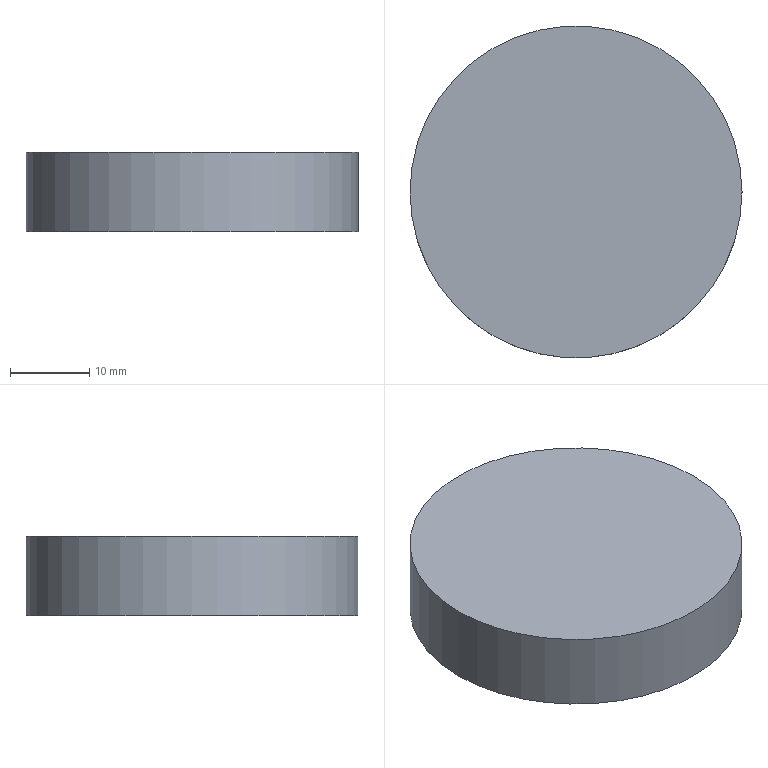Component | NX | CH3404_1-3 | 1 solid | 3 faces | box 42 x 42 x 10 mm | volume 13854 mm3 | plane 2 | cylinder 1 | commonest cylinder face diameters 42 x1
STEP:
#1=CARTESIAN_POINT('',(0.,0.,0.));
#2=DIRECTION('',(0.,0.,1.));
#3=DIRECTION('',(1.,0.,0.));
#4=AXIS2_PLACEMENT_3D('',#1,#2,#3);
#5=CARTESIAN_POINT('',(21.,0.,10.));
#6=VERTEX_POINT('',#5);
#7=CARTESIAN_POINT('',(0.,0.,10.));
#8=DIRECTION('',(0.,0.,1.));
#9=DIRECTION('',(1.,0.,0.));
#10=AXIS2_PLACEMENT_3D('',#7,#8,#9);
#11=CIRCLE('',#10,21.);
#12=CARTESIAN_POINT('',(0.,0.,10.));
#13=DIRECTION('',(0.,0.,-1.));
#14=DIRECTION('',(-1.,0.,0.));
#15=AXIS2_PLACEMENT_3D('',#12,#13,#14);
#16=CYLINDRICAL_SURFACE('',#15,21.);
#17=CARTESIAN_POINT('',(9.425,0.));
#18=DIRECTION('',(-1.,0.));
#19=VECTOR('',#18,1.);
#20=LINE('',#17,#19);
#21=(GEOMETRIC_REPRESENTATION_CONTEXT(2)PARAMETRIC_REPRESENTATION_CONTEXT()REPRESENTATION_CONTEXT('',''));
#22=DEFINITIONAL_REPRESENTATION('',(#20),#21);
#23=PCURVE('',#16,#22);
#24=CARTESIAN_POINT('',(0.,0.,10.));
#25=DIRECTION('',(0.,0.,1.));
#26=DIRECTION('',(1.,0.,0.));
#27=AXIS2_PLACEMENT_3D('',#24,#25,#26);
#28=PLANE('',#27);
#29=CARTESIAN_POINT('',(0.,0.));
#30=DIRECTION('',(1.,0.));
#31=AXIS2_PLACEMENT_2D('',#29,#30);
#32=CIRCLE('',#31,21.);
#33=(GEOMETRIC_REPRESENTATION_CONTEXT(2)PARAMETRIC_REPRESENTATION_CONTEXT()REPRESENTATION_CONTEXT('',''));
#34=DEFINITIONAL_REPRESENTATION('',(#32),#33);
#35=PCURVE('',#28,#34);
#36=SURFACE_CURVE('',#11,(#23,#35),.PCURVE_S1.);
#37=EDGE_CURVE('',#6,#6,#36,.T.);
#38=ORIENTED_EDGE('',*,*,#37,.F.);
#39=CARTESIAN_POINT('',(21.,0.,0.));
#40=VERTEX_POINT('',#39);
#41=CARTESIAN_POINT('',(21.,0.,10.));
#42=CARTESIAN_POINT('',(21.,0.,0.));
#43=B_SPLINE_CURVE_WITH_KNOTS('',1,(#41,#42),.UNSPECIFIED.,.F.,.F.,(2,2),(0.,10.),.PIECEWISE_BEZIER_KNOTS.);
#44=CARTESIAN_POINT('',(9.425,0.));
#45=DIRECTION('',(0.,1.));
#46=VECTOR('',#45,1.);
#47=LINE('',#44,#46);
#48=(GEOMETRIC_REPRESENTATION_CONTEXT(2)PARAMETRIC_REPRESENTATION_CONTEXT()REPRESENTATION_CONTEXT('',''));
#49=DEFINITIONAL_REPRESENTATION('',(#47),#48);
#50=PCURVE('',#16,#49);
#51=CARTESIAN_POINT('',(3.142,0.));
#52=DIRECTION('',(0.,1.));
#53=VECTOR('',#52,1.);
#54=LINE('',#51,#53);
#55=(GEOMETRIC_REPRESENTATION_CONTEXT(2)PARAMETRIC_REPRESENTATION_CONTEXT()REPRESENTATION_CONTEXT('',''));
#56=DEFINITIONAL_REPRESENTATION('',(#54),#55);
#57=PCURVE('',#16,#56);
#58=SEAM_CURVE('',#43,(#50,#57),.PCURVE_S1.);
#59=EDGE_CURVE('',#6,#40,#58,.T.);
#60=ORIENTED_EDGE('',*,*,#59,.T.);
#61=CARTESIAN_POINT('',(0.,0.,0.));
#62=DIRECTION('',(0.,0.,1.));
#63=DIRECTION('',(1.,0.,0.));
#64=AXIS2_PLACEMENT_3D('',#61,#62,#63);
#65=CIRCLE('',#64,21.);
#66=CARTESIAN_POINT('',(9.425,10.));
#67=DIRECTION('',(-1.,0.));
#68=VECTOR('',#67,1.);
#69=LINE('',#66,#68);
#70=(GEOMETRIC_REPRESENTATION_CONTEXT(2)PARAMETRIC_REPRESENTATION_CONTEXT()REPRESENTATION_CONTEXT('',''));
#71=DEFINITIONAL_REPRESENTATION('',(#69),#70);
#72=PCURVE('',#16,#71);
#73=CARTESIAN_POINT('',(0.,0.,0.));
#74=DIRECTION('',(0.,0.,1.));
#75=DIRECTION('',(1.,0.,0.));
#76=AXIS2_PLACEMENT_3D('',#73,#74,#75);
#77=PLANE('',#76);
#78=CARTESIAN_POINT('',(0.,0.));
#79=DIRECTION('',(1.,0.));
#80=AXIS2_PLACEMENT_2D('',#78,#79);
#81=CIRCLE('',#80,21.);
#82=(GEOMETRIC_REPRESENTATION_CONTEXT(2)PARAMETRIC_REPRESENTATION_CONTEXT()REPRESENTATION_CONTEXT('',''));
#83=DEFINITIONAL_REPRESENTATION('',(#81),#82);
#84=PCURVE('',#77,#83);
#85=SURFACE_CURVE('',#65,(#72,#84),.PCURVE_S1.);
#86=EDGE_CURVE('',#40,#40,#85,.T.);
#87=ORIENTED_EDGE('',*,*,#86,.T.);
#88=ORIENTED_EDGE('',*,*,#59,.F.);
#89=EDGE_LOOP('',(#38,#60,#87,#88));
#90=FACE_BOUND('',#89,.T.);
#91=ADVANCED_FACE('',(#90),#16,.T.);
#92=ORIENTED_EDGE('',*,*,#37,.T.);
#93=EDGE_LOOP('',(#92));
#94=FACE_BOUND('',#93,.T.);
#95=ADVANCED_FACE('',(#94),#28,.T.);
#96=ORIENTED_EDGE('',*,*,#86,.F.);
#97=EDGE_LOOP('',(#96));
#98=FACE_BOUND('',#97,.T.);
#99=ADVANCED_FACE('',(#98),#77,.F.);
#100=CLOSED_SHELL('',(#91,#95,#99));
#101=MANIFOLD_SOLID_BREP('',#100);
#102=(LENGTH_UNIT()NAMED_UNIT(*)SI_UNIT(.MILLI.,.METRE.));
#103=UNCERTAINTY_MEASURE_WITH_UNIT(LENGTH_MEASURE(0.00001),#102,'','');
#104=(NAMED_UNIT(*)PLANE_ANGLE_UNIT()SI_UNIT($,.RADIAN.));
#105=(NAMED_UNIT(*)SI_UNIT($,.STERADIAN.)SOLID_ANGLE_UNIT());
#106=(GEOMETRIC_REPRESENTATION_CONTEXT(3)GLOBAL_UNCERTAINTY_ASSIGNED_CONTEXT((#103))GLOBAL_UNIT_ASSIGNED_CONTEXT((#102,#104,#105))REPRESENTATION_CONTEXT('',''));
#107=ADVANCED_BREP_SHAPE_REPRESENTATION('',(#4,#101),#106);